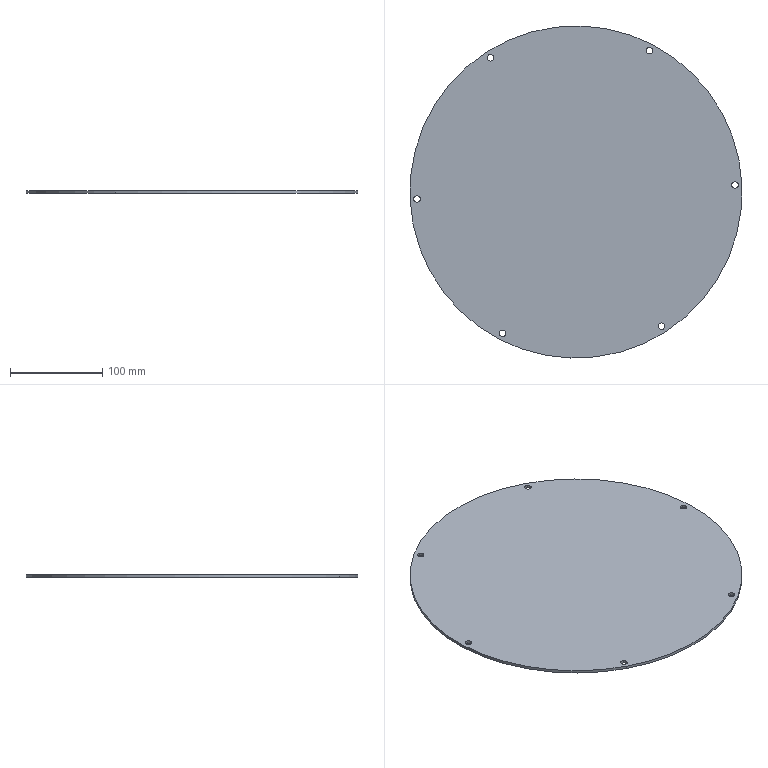Component | SolidWorks | YC1-250-02-21CrankshaftEndCover-1 | 1 solid | 16 faces | box 360 x 360 x 3 mm | volume 304670 mm3 | cylinder 14 | plane 2 | commonest cylinder face diameters 7 x12 360 x2 | material Plain Carbon Steel
STEP:
#1=COLOUR_RGB('',0.7922,0.8196,0.9333);
#2=FILL_AREA_STYLE_COLOUR('',#1);
#3=FILL_AREA_STYLE('',(#2));
#4=SURFACE_STYLE_FILL_AREA(#3);
#5=SURFACE_SIDE_STYLE('',(#4));
#6=SURFACE_STYLE_USAGE(.BOTH.,#5);
#7=PRESENTATION_STYLE_ASSIGNMENT((#6));
#8=CARTESIAN_POINT('',(-3.267,125.404,18.425));
#9=VERTEX_POINT('',#8);
#10=CARTESIAN_POINT('',(3.267,137.982,18.425));
#11=VERTEX_POINT('',#10);
#12=CARTESIAN_POINT('',(0.,131.693,18.425));
#13=DIRECTION('',(0.,0.,1.));
#14=DIRECTION('',(0.461,0.8874,0.));
#15=AXIS2_PLACEMENT_3D('',#12,#13,#14);
#16=CIRCLE('',#15,7.087);
#17=EDGE_CURVE('',#9,#11,#16,.T.);
#18=ORIENTED_EDGE('',*,*,#17,.F.);
#19=CARTESIAN_POINT('',(-3.267,125.404,18.307));
#20=VERTEX_POINT('',#19);
#21=CARTESIAN_POINT('',(-3.267,125.404,18.425));
#22=DIRECTION('',(0.,0.,-1.));
#23=VECTOR('',#22,39.37);
#24=LINE('',#21,#23);
#25=EDGE_CURVE('',#9,#20,#24,.T.);
#26=ORIENTED_EDGE('',*,*,#25,.T.);
#27=CARTESIAN_POINT('',(3.267,137.982,18.307));
#28=VERTEX_POINT('',#27);
#29=CARTESIAN_POINT('',(0.,131.693,18.307));
#30=DIRECTION('',(0.,0.,1.));
#31=DIRECTION('',(0.461,0.8874,0.));
#32=AXIS2_PLACEMENT_3D('',#29,#30,#31);
#33=CIRCLE('',#32,7.087);
#34=EDGE_CURVE('',#20,#28,#33,.T.);
#35=ORIENTED_EDGE('',*,*,#34,.T.);
#36=CARTESIAN_POINT('',(3.267,137.982,18.425));
#37=DIRECTION('',(0.,0.,-1.));
#38=VECTOR('',#37,39.37);
#39=LINE('',#36,#38);
#40=EDGE_CURVE('',#11,#28,#39,.T.);
#41=ORIENTED_EDGE('',*,*,#40,.F.);
#42=EDGE_LOOP('',(#18,#26,#35,#41));
#43=FACE_OUTER_BOUND('',#42,.T.);
#44=CARTESIAN_POINT('',(0.,131.693,18.425));
#45=DIRECTION('',(0.,0.,-1.));
#46=DIRECTION('',(0.461,0.8874,0.));
#47=AXIS2_PLACEMENT_3D('',#44,#45,#46);
#48=CYLINDRICAL_SURFACE('',#47,7.087);
#49=ADVANCED_FACE('',(#43),#48,.T.);
#50=CARTESIAN_POINT('',(-3.067,125.788,18.307));
#51=VERTEX_POINT('',#50);
#52=CARTESIAN_POINT('',(-3.194,125.544,18.307));
#53=VERTEX_POINT('',#52);
#54=CARTESIAN_POINT('',(-3.131,125.666,18.307));
#55=DIRECTION('',(0.,0.,1.));
#56=DIRECTION('',(-0.461,-0.8874,0.));
#57=AXIS2_PLACEMENT_3D('',#54,#55,#56);
#58=CIRCLE('',#57,0.1378);
#59=EDGE_CURVE('',#51,#53,#58,.T.);
#60=ORIENTED_EDGE('',*,*,#59,.F.);
#61=CARTESIAN_POINT('',(-3.067,125.788,18.425));
#62=VERTEX_POINT('',#61);
#63=CARTESIAN_POINT('',(-3.067,125.788,18.425));
#64=DIRECTION('',(0.,0.,1.));
#65=VECTOR('',#64,39.37);
#66=LINE('',#63,#65);
#67=EDGE_CURVE('',#51,#62,#66,.T.);
#68=ORIENTED_EDGE('',*,*,#67,.T.);
#69=CARTESIAN_POINT('',(-3.194,125.544,18.425));
#70=VERTEX_POINT('',#69);
#71=CARTESIAN_POINT('',(-3.131,125.666,18.425));
#72=DIRECTION('',(0.,0.,-1.));
#73=DIRECTION('',(-0.461,-0.8874,0.));
#74=AXIS2_PLACEMENT_3D('',#71,#72,#73);
#75=CIRCLE('',#74,0.1378);
#76=EDGE_CURVE('',#70,#62,#75,.T.);
#77=ORIENTED_EDGE('',*,*,#76,.F.);
#78=CARTESIAN_POINT('',(-3.194,125.544,18.425));
#79=DIRECTION('',(0.,0.,1.));
#80=VECTOR('',#79,39.37);
#81=LINE('',#78,#80);
#82=EDGE_CURVE('',#53,#70,#81,.T.);
#83=ORIENTED_EDGE('',*,*,#82,.F.);
#84=EDGE_LOOP('',(#60,#68,#77,#83));
#85=FACE_OUTER_BOUND('',#84,.T.);
#86=CARTESIAN_POINT('',(-3.131,125.666,18.425));
#87=DIRECTION('',(0.,0.,1.));
#88=DIRECTION('',(-0.461,-0.8874,0.));
#89=AXIS2_PLACEMENT_3D('',#86,#87,#88);
#90=CYLINDRICAL_SURFACE('',#89,0.1378);
#91=ADVANCED_FACE('',(#85),#90,.F.);
#92=CARTESIAN_POINT('',(-6.721,131.513,18.307));
#93=VERTEX_POINT('',#92);
#94=CARTESIAN_POINT('',(-6.848,131.268,18.307));
#95=VERTEX_POINT('',#94);
#96=CARTESIAN_POINT('',(-6.785,131.391,18.307));
#97=DIRECTION('',(0.,0.,1.));
#98=DIRECTION('',(-0.461,-0.8874,0.));
#99=AXIS2_PLACEMENT_3D('',#96,#97,#98);
#100=CIRCLE('',#99,0.1378);
#101=EDGE_CURVE('',#93,#95,#100,.T.);
#102=ORIENTED_EDGE('',*,*,#101,.F.);
#103=CARTESIAN_POINT('',(-6.721,131.513,18.425));
#104=VERTEX_POINT('',#103);
#105=CARTESIAN_POINT('',(-6.721,131.513,18.425));
#106=DIRECTION('',(0.,0.,1.));
#107=VECTOR('',#106,39.37);
#108=LINE('',#105,#107);
#109=EDGE_CURVE('',#93,#104,#108,.T.);
#110=ORIENTED_EDGE('',*,*,#109,.T.);
#111=CARTESIAN_POINT('',(-6.848,131.268,18.425));
#112=VERTEX_POINT('',#111);
#113=CARTESIAN_POINT('',(-6.785,131.391,18.425));
#114=DIRECTION('',(0.,0.,-1.));
#115=DIRECTION('',(-0.461,-0.8874,0.));
#116=AXIS2_PLACEMENT_3D('',#113,#114,#115);
#117=CIRCLE('',#116,0.1378);
#118=EDGE_CURVE('',#112,#104,#117,.T.);
#119=ORIENTED_EDGE('',*,*,#118,.F.);
#120=CARTESIAN_POINT('',(-6.848,131.268,18.425));
#121=DIRECTION('',(0.,0.,1.));
#122=VECTOR('',#121,39.37);
#123=LINE('',#120,#122);
#124=EDGE_CURVE('',#95,#112,#123,.T.);
#125=ORIENTED_EDGE('',*,*,#124,.F.);
#126=EDGE_LOOP('',(#102,#110,#119,#125));
#127=FACE_OUTER_BOUND('',#126,.T.);
#128=CARTESIAN_POINT('',(-6.785,131.391,18.425));
#129=DIRECTION('',(0.,0.,1.));
#130=DIRECTION('',(-0.461,-0.8874,0.));
#131=AXIS2_PLACEMENT_3D('',#128,#129,#130);
#132=CYLINDRICAL_SURFACE('',#131,0.1378);
#133=ADVANCED_FACE('',(#127),#132,.F.);
#134=CARTESIAN_POINT('',(-3.591,137.54,18.307));
#135=VERTEX_POINT('',#134);
#136=CARTESIAN_POINT('',(-3.718,137.295,18.307));
#137=VERTEX_POINT('',#136);
#138=CARTESIAN_POINT('',(-3.654,137.417,18.307));
#139=DIRECTION('',(0.,0.,1.));
#140=DIRECTION('',(-0.461,-0.8874,0.));
#141=AXIS2_PLACEMENT_3D('',#138,#139,#140);
#142=CIRCLE('',#141,0.1378);
#143=EDGE_CURVE('',#135,#137,#142,.T.);
#144=ORIENTED_EDGE('',*,*,#143,.F.);
#145=CARTESIAN_POINT('',(-3.591,137.54,18.425));
#146=VERTEX_POINT('',#145);
#147=CARTESIAN_POINT('',(-3.591,137.54,18.425));
#148=DIRECTION('',(0.,0.,1.));
#149=VECTOR('',#148,39.37);
#150=LINE('',#147,#149);
#151=EDGE_CURVE('',#135,#146,#150,.T.);
#152=ORIENTED_EDGE('',*,*,#151,.T.);
#153=CARTESIAN_POINT('',(-3.718,137.295,18.425));
#154=VERTEX_POINT('',#153);
#155=CARTESIAN_POINT('',(-3.654,137.417,18.425));
#156=DIRECTION('',(0.,0.,-1.));
#157=DIRECTION('',(-0.461,-0.8874,0.));
#158=AXIS2_PLACEMENT_3D('',#155,#156,#157);
#159=CIRCLE('',#158,0.1378);
#160=EDGE_CURVE('',#154,#146,#159,.T.);
#161=ORIENTED_EDGE('',*,*,#160,.F.);
#162=CARTESIAN_POINT('',(-3.718,137.295,18.425));
#163=DIRECTION('',(0.,0.,1.));
#164=VECTOR('',#163,39.37);
#165=LINE('',#162,#164);
#166=EDGE_CURVE('',#137,#154,#165,.T.);
#167=ORIENTED_EDGE('',*,*,#166,.F.);
#168=EDGE_LOOP('',(#144,#152,#161,#167));
#169=FACE_OUTER_BOUND('',#168,.T.);
#170=CARTESIAN_POINT('',(-3.654,137.417,18.425));
#171=DIRECTION('',(0.,0.,1.));
#172=DIRECTION('',(-0.461,-0.8874,0.));
#173=AXIS2_PLACEMENT_3D('',#170,#171,#172);
#174=CYLINDRICAL_SURFACE('',#173,0.1378);
#175=ADVANCED_FACE('',(#169),#174,.F.);
#176=CARTESIAN_POINT('',(3.194,137.842,18.307));
#177=VERTEX_POINT('',#176);
#178=CARTESIAN_POINT('',(3.067,137.597,18.307));
#179=VERTEX_POINT('',#178);
#180=CARTESIAN_POINT('',(3.131,137.72,18.307));
#181=DIRECTION('',(0.,0.,1.));
#182=DIRECTION('',(-0.461,-0.8874,0.));
#183=AXIS2_PLACEMENT_3D('',#180,#181,#182);
#184=CIRCLE('',#183,0.1378);
#185=EDGE_CURVE('',#177,#179,#184,.T.);
#186=ORIENTED_EDGE('',*,*,#185,.F.);
#187=CARTESIAN_POINT('',(3.194,137.842,18.425));
#188=VERTEX_POINT('',#187);
#189=CARTESIAN_POINT('',(3.194,137.842,18.425));
#190=DIRECTION('',(0.,0.,1.));
#191=VECTOR('',#190,39.37);
#192=LINE('',#189,#191);
#193=EDGE_CURVE('',#177,#188,#192,.T.);
#194=ORIENTED_EDGE('',*,*,#193,.T.);
#195=CARTESIAN_POINT('',(3.067,137.597,18.425));
#196=VERTEX_POINT('',#195);
#197=CARTESIAN_POINT('',(3.131,137.72,18.425));
#198=DIRECTION('',(0.,0.,-1.));
#199=DIRECTION('',(-0.461,-0.8874,0.));
#200=AXIS2_PLACEMENT_3D('',#197,#198,#199);
#201=CIRCLE('',#200,0.1378);
#202=EDGE_CURVE('',#196,#188,#201,.T.);
#203=ORIENTED_EDGE('',*,*,#202,.F.);
#204=CARTESIAN_POINT('',(3.067,137.597,18.425));
#205=DIRECTION('',(0.,0.,1.));
#206=VECTOR('',#205,39.37);
#207=LINE('',#204,#206);
#208=EDGE_CURVE('',#179,#196,#207,.T.);
#209=ORIENTED_EDGE('',*,*,#208,.F.);
#210=EDGE_LOOP('',(#186,#194,#203,#209));
#211=FACE_OUTER_BOUND('',#210,.T.);
#212=CARTESIAN_POINT('',(3.131,137.72,18.425));
#213=DIRECTION('',(0.,0.,1.));
#214=DIRECTION('',(-0.461,-0.8874,0.));
#215=AXIS2_PLACEMENT_3D('',#212,#213,#214);
#216=CYLINDRICAL_SURFACE('',#215,0.1378);
#217=ADVANCED_FACE('',(#211),#216,.F.);
#218=CARTESIAN_POINT('',(6.848,132.117,18.307));
#219=VERTEX_POINT('',#218);
#220=CARTESIAN_POINT('',(6.721,131.873,18.307));
#221=VERTEX_POINT('',#220);
#222=CARTESIAN_POINT('',(6.785,131.995,18.307));
#223=DIRECTION('',(0.,0.,1.));
#224=DIRECTION('',(-0.461,-0.8874,0.));
#225=AXIS2_PLACEMENT_3D('',#222,#223,#224);
#226=CIRCLE('',#225,0.1378);
#227=EDGE_CURVE('',#219,#221,#226,.T.);
#228=ORIENTED_EDGE('',*,*,#227,.F.);
#229=CARTESIAN_POINT('',(6.848,132.117,18.425));
#230=VERTEX_POINT('',#229);
#231=CARTESIAN_POINT('',(6.848,132.117,18.425));
#232=DIRECTION('',(0.,0.,1.));
#233=VECTOR('',#232,39.37);
#234=LINE('',#231,#233);
#235=EDGE_CURVE('',#219,#230,#234,.T.);
#236=ORIENTED_EDGE('',*,*,#235,.T.);
#237=CARTESIAN_POINT('',(6.721,131.873,18.425));
#238=VERTEX_POINT('',#237);
#239=CARTESIAN_POINT('',(6.785,131.995,18.425));
#240=DIRECTION('',(0.,0.,-1.));
#241=DIRECTION('',(-0.461,-0.8874,0.));
#242=AXIS2_PLACEMENT_3D('',#239,#240,#241);
#243=CIRCLE('',#242,0.1378);
#244=EDGE_CURVE('',#238,#230,#243,.T.);
#245=ORIENTED_EDGE('',*,*,#244,.F.);
#246=CARTESIAN_POINT('',(6.721,131.873,18.425));
#247=DIRECTION('',(0.,0.,1.));
#248=VECTOR('',#247,39.37);
#249=LINE('',#246,#248);
#250=EDGE_CURVE('',#221,#238,#249,.T.);
#251=ORIENTED_EDGE('',*,*,#250,.F.);
#252=EDGE_LOOP('',(#228,#236,#245,#251));
#253=FACE_OUTER_BOUND('',#252,.T.);
#254=CARTESIAN_POINT('',(6.785,131.995,18.425));
#255=DIRECTION('',(0.,0.,1.));
#256=DIRECTION('',(-0.461,-0.8874,0.));
#257=AXIS2_PLACEMENT_3D('',#254,#255,#256);
#258=CYLINDRICAL_SURFACE('',#257,0.1378);
#259=ADVANCED_FACE('',(#253),#258,.F.);
#260=CARTESIAN_POINT('',(3.718,126.091,18.307));
#261=VERTEX_POINT('',#260);
#262=CARTESIAN_POINT('',(3.591,125.846,18.307));
#263=VERTEX_POINT('',#262);
#264=CARTESIAN_POINT('',(3.654,125.968,18.307));
#265=DIRECTION('',(0.,0.,1.));
#266=DIRECTION('',(-0.461,-0.8874,0.));
#267=AXIS2_PLACEMENT_3D('',#264,#265,#266);
#268=CIRCLE('',#267,0.1378);
#269=EDGE_CURVE('',#261,#263,#268,.T.);
#270=ORIENTED_EDGE('',*,*,#269,.F.);
#271=CARTESIAN_POINT('',(3.718,126.091,18.425));
#272=VERTEX_POINT('',#271);
#273=CARTESIAN_POINT('',(3.718,126.091,18.425));
#274=DIRECTION('',(0.,0.,1.));
#275=VECTOR('',#274,39.37);
#276=LINE('',#273,#275);
#277=EDGE_CURVE('',#261,#272,#276,.T.);
#278=ORIENTED_EDGE('',*,*,#277,.T.);
#279=CARTESIAN_POINT('',(3.591,125.846,18.425));
#280=VERTEX_POINT('',#279);
#281=CARTESIAN_POINT('',(3.654,125.968,18.425));
#282=DIRECTION('',(0.,0.,-1.));
#283=DIRECTION('',(-0.461,-0.8874,0.));
#284=AXIS2_PLACEMENT_3D('',#281,#282,#283);
#285=CIRCLE('',#284,0.1378);
#286=EDGE_CURVE('',#280,#272,#285,.T.);
#287=ORIENTED_EDGE('',*,*,#286,.F.);
#288=CARTESIAN_POINT('',(3.591,125.846,18.425));
#289=DIRECTION('',(0.,0.,1.));
#290=VECTOR('',#289,39.37);
#291=LINE('',#288,#290);
#292=EDGE_CURVE('',#263,#280,#291,.T.);
#293=ORIENTED_EDGE('',*,*,#292,.F.);
#294=EDGE_LOOP('',(#270,#278,#287,#293));
#295=FACE_OUTER_BOUND('',#294,.T.);
#296=CARTESIAN_POINT('',(3.654,125.968,18.425));
#297=DIRECTION('',(0.,0.,1.));
#298=DIRECTION('',(-0.461,-0.8874,0.));
#299=AXIS2_PLACEMENT_3D('',#296,#297,#298);
#300=CYLINDRICAL_SURFACE('',#299,0.1378);
#301=ADVANCED_FACE('',(#295),#300,.F.);
#302=CARTESIAN_POINT('',(0.,131.693,18.425));
#303=DIRECTION('',(0.,0.,1.));
#304=DIRECTION('',(0.461,0.8874,0.));
#305=AXIS2_PLACEMENT_3D('',#302,#303,#304);
#306=CIRCLE('',#305,7.087);
#307=EDGE_CURVE('',#11,#9,#306,.T.);
#308=ORIENTED_EDGE('',*,*,#307,.T.);
#309=ORIENTED_EDGE('',*,*,#17,.T.);
#310=EDGE_LOOP('',(#308,#309));
#311=FACE_OUTER_BOUND('',#310,.T.);
#312=ORIENTED_EDGE('',*,*,#76,.T.);
#313=CARTESIAN_POINT('',(-3.131,125.666,18.425));
#314=DIRECTION('',(0.,0.,-1.));
#315=DIRECTION('',(-0.461,-0.8874,0.));
#316=AXIS2_PLACEMENT_3D('',#313,#314,#315);
#317=CIRCLE('',#316,0.1378);
#318=EDGE_CURVE('',#62,#70,#317,.T.);
#319=ORIENTED_EDGE('',*,*,#318,.T.);
#320=EDGE_LOOP('',(#312,#319));
#321=FACE_BOUND('',#320,.T.);
#322=ORIENTED_EDGE('',*,*,#118,.T.);
#323=CARTESIAN_POINT('',(-6.785,131.391,18.425));
#324=DIRECTION('',(0.,0.,-1.));
#325=DIRECTION('',(-0.461,-0.8874,0.));
#326=AXIS2_PLACEMENT_3D('',#323,#324,#325);
#327=CIRCLE('',#326,0.1378);
#328=EDGE_CURVE('',#104,#112,#327,.T.);
#329=ORIENTED_EDGE('',*,*,#328,.T.);
#330=EDGE_LOOP('',(#322,#329));
#331=FACE_BOUND('',#330,.T.);
#332=ORIENTED_EDGE('',*,*,#160,.T.);
#333=CARTESIAN_POINT('',(-3.654,137.417,18.425));
#334=DIRECTION('',(0.,0.,-1.));
#335=DIRECTION('',(-0.461,-0.8874,0.));
#336=AXIS2_PLACEMENT_3D('',#333,#334,#335);
#337=CIRCLE('',#336,0.1378);
#338=EDGE_CURVE('',#146,#154,#337,.T.);
#339=ORIENTED_EDGE('',*,*,#338,.T.);
#340=EDGE_LOOP('',(#332,#339));
#341=FACE_BOUND('',#340,.T.);
#342=ORIENTED_EDGE('',*,*,#202,.T.);
#343=CARTESIAN_POINT('',(3.131,137.72,18.425));
#344=DIRECTION('',(0.,0.,-1.));
#345=DIRECTION('',(-0.461,-0.8874,0.));
#346=AXIS2_PLACEMENT_3D('',#343,#344,#345);
#347=CIRCLE('',#346,0.1378);
#348=EDGE_CURVE('',#188,#196,#347,.T.);
#349=ORIENTED_EDGE('',*,*,#348,.T.);
#350=EDGE_LOOP('',(#342,#349));
#351=FACE_BOUND('',#350,.T.);
#352=ORIENTED_EDGE('',*,*,#244,.T.);
#353=CARTESIAN_POINT('',(6.785,131.995,18.425));
#354=DIRECTION('',(0.,0.,-1.));
#355=DIRECTION('',(-0.461,-0.8874,0.));
#356=AXIS2_PLACEMENT_3D('',#353,#354,#355);
#357=CIRCLE('',#356,0.1378);
#358=EDGE_CURVE('',#230,#238,#357,.T.);
#359=ORIENTED_EDGE('',*,*,#358,.T.);
#360=EDGE_LOOP('',(#352,#359));
#361=FACE_BOUND('',#360,.T.);
#362=ORIENTED_EDGE('',*,*,#286,.T.);
#363=CARTESIAN_POINT('',(3.654,125.968,18.425));
#364=DIRECTION('',(0.,0.,-1.));
#365=DIRECTION('',(-0.461,-0.8874,0.));
#366=AXIS2_PLACEMENT_3D('',#363,#364,#365);
#367=CIRCLE('',#366,0.1378);
#368=EDGE_CURVE('',#272,#280,#367,.T.);
#369=ORIENTED_EDGE('',*,*,#368,.T.);
#370=EDGE_LOOP('',(#362,#369));
#371=FACE_BOUND('',#370,.T.);
#372=CARTESIAN_POINT('',(0.,131.693,18.425));
#373=DIRECTION('',(0.,0.,1.));
#374=DIRECTION('',(-0.461,-0.8874,0.));
#375=AXIS2_PLACEMENT_3D('',#372,#373,#374);
#376=PLANE('',#375);
#377=ADVANCED_FACE('',(#311,#321,#331,#341,#351,#361,#371),#376,.T.);
#378=ORIENTED_EDGE('',*,*,#25,.F.);
#379=ORIENTED_EDGE('',*,*,#307,.F.);
#380=ORIENTED_EDGE('',*,*,#40,.T.);
#381=CARTESIAN_POINT('',(0.,131.693,18.307));
#382=DIRECTION('',(0.,0.,1.));
#383=DIRECTION('',(0.461,0.8874,0.));
#384=AXIS2_PLACEMENT_3D('',#381,#382,#383);
#385=CIRCLE('',#384,7.087);
#386=EDGE_CURVE('',#28,#20,#385,.T.);
#387=ORIENTED_EDGE('',*,*,#386,.T.);
#388=EDGE_LOOP('',(#378,#379,#380,#387));
#389=FACE_OUTER_BOUND('',#388,.T.);
#390=CARTESIAN_POINT('',(0.,131.693,18.425));
#391=DIRECTION('',(0.,0.,-1.));
#392=DIRECTION('',(0.461,0.8874,0.));
#393=AXIS2_PLACEMENT_3D('',#390,#391,#392);
#394=CYLINDRICAL_SURFACE('',#393,7.087);
#395=ADVANCED_FACE('',(#389),#394,.T.);
#396=ORIENTED_EDGE('',*,*,#67,.F.);
#397=CARTESIAN_POINT('',(-3.131,125.666,18.307));
#398=DIRECTION('',(0.,0.,1.));
#399=DIRECTION('',(-0.461,-0.8874,0.));
#400=AXIS2_PLACEMENT_3D('',#397,#398,#399);
#401=CIRCLE('',#400,0.1378);
#402=EDGE_CURVE('',#53,#51,#401,.T.);
#403=ORIENTED_EDGE('',*,*,#402,.F.);
#404=ORIENTED_EDGE('',*,*,#82,.T.);
#405=ORIENTED_EDGE('',*,*,#318,.F.);
#406=EDGE_LOOP('',(#396,#403,#404,#405));
#407=FACE_OUTER_BOUND('',#406,.T.);
#408=CARTESIAN_POINT('',(-3.131,125.666,18.425));
#409=DIRECTION('',(0.,0.,1.));
#410=DIRECTION('',(-0.461,-0.8874,0.));
#411=AXIS2_PLACEMENT_3D('',#408,#409,#410);
#412=CYLINDRICAL_SURFACE('',#411,0.1378);
#413=ADVANCED_FACE('',(#407),#412,.F.);
#414=ORIENTED_EDGE('',*,*,#109,.F.);
#415=CARTESIAN_POINT('',(-6.785,131.391,18.307));
#416=DIRECTION('',(0.,0.,1.));
#417=DIRECTION('',(-0.461,-0.8874,0.));
#418=AXIS2_PLACEMENT_3D('',#415,#416,#417);
#419=CIRCLE('',#418,0.1378);
#420=EDGE_CURVE('',#95,#93,#419,.T.);
#421=ORIENTED_EDGE('',*,*,#420,.F.);
#422=ORIENTED_EDGE('',*,*,#124,.T.);
#423=ORIENTED_EDGE('',*,*,#328,.F.);
#424=EDGE_LOOP('',(#414,#421,#422,#423));
#425=FACE_OUTER_BOUND('',#424,.T.);
#426=CARTESIAN_POINT('',(-6.785,131.391,18.425));
#427=DIRECTION('',(0.,0.,1.));
#428=DIRECTION('',(-0.461,-0.8874,0.));
#429=AXIS2_PLACEMENT_3D('',#426,#427,#428);
#430=CYLINDRICAL_SURFACE('',#429,0.1378);
#431=ADVANCED_FACE('',(#425),#430,.F.);
#432=ORIENTED_EDGE('',*,*,#151,.F.);
#433=CARTESIAN_POINT('',(-3.654,137.417,18.307));
#434=DIRECTION('',(0.,0.,1.));
#435=DIRECTION('',(-0.461,-0.8874,0.));
#436=AXIS2_PLACEMENT_3D('',#433,#434,#435);
#437=CIRCLE('',#436,0.1378);
#438=EDGE_CURVE('',#137,#135,#437,.T.);
#439=ORIENTED_EDGE('',*,*,#438,.F.);
#440=ORIENTED_EDGE('',*,*,#166,.T.);
#441=ORIENTED_EDGE('',*,*,#338,.F.);
#442=EDGE_LOOP('',(#432,#439,#440,#441));
#443=FACE_OUTER_BOUND('',#442,.T.);
#444=CARTESIAN_POINT('',(-3.654,137.417,18.425));
#445=DIRECTION('',(0.,0.,1.));
#446=DIRECTION('',(-0.461,-0.8874,0.));
#447=AXIS2_PLACEMENT_3D('',#444,#445,#446);
#448=CYLINDRICAL_SURFACE('',#447,0.1378);
#449=ADVANCED_FACE('',(#443),#448,.F.);
#450=ORIENTED_EDGE('',*,*,#193,.F.);
#451=CARTESIAN_POINT('',(3.131,137.72,18.307));
#452=DIRECTION('',(0.,0.,1.));
#453=DIRECTION('',(-0.461,-0.8874,0.));
#454=AXIS2_PLACEMENT_3D('',#451,#452,#453);
#455=CIRCLE('',#454,0.1378);
#456=EDGE_CURVE('',#179,#177,#455,.T.);
#457=ORIENTED_EDGE('',*,*,#456,.F.);
#458=ORIENTED_EDGE('',*,*,#208,.T.);
#459=ORIENTED_EDGE('',*,*,#348,.F.);
#460=EDGE_LOOP('',(#450,#457,#458,#459));
#461=FACE_OUTER_BOUND('',#460,.T.);
#462=CARTESIAN_POINT('',(3.131,137.72,18.425));
#463=DIRECTION('',(0.,0.,1.));
#464=DIRECTION('',(-0.461,-0.8874,0.));
#465=AXIS2_PLACEMENT_3D('',#462,#463,#464);
#466=CYLINDRICAL_SURFACE('',#465,0.1378);
#467=ADVANCED_FACE('',(#461),#466,.F.);
#468=ORIENTED_EDGE('',*,*,#235,.F.);
#469=CARTESIAN_POINT('',(6.785,131.995,18.307));
#470=DIRECTION('',(0.,0.,1.));
#471=DIRECTION('',(-0.461,-0.8874,0.));
#472=AXIS2_PLACEMENT_3D('',#469,#470,#471);
#473=CIRCLE('',#472,0.1378);
#474=EDGE_CURVE('',#221,#219,#473,.T.);
#475=ORIENTED_EDGE('',*,*,#474,.F.);
#476=ORIENTED_EDGE('',*,*,#250,.T.);
#477=ORIENTED_EDGE('',*,*,#358,.F.);
#478=EDGE_LOOP('',(#468,#475,#476,#477));
#479=FACE_OUTER_BOUND('',#478,.T.);
#480=CARTESIAN_POINT('',(6.785,131.995,18.425));
#481=DIRECTION('',(0.,0.,1.));
#482=DIRECTION('',(-0.461,-0.8874,0.));
#483=AXIS2_PLACEMENT_3D('',#480,#481,#482);
#484=CYLINDRICAL_SURFACE('',#483,0.1378);
#485=ADVANCED_FACE('',(#479),#484,.F.);
#486=ORIENTED_EDGE('',*,*,#277,.F.);
#487=CARTESIAN_POINT('',(3.654,125.968,18.307));
#488=DIRECTION('',(0.,0.,1.));
#489=DIRECTION('',(-0.461,-0.8874,0.));
#490=AXIS2_PLACEMENT_3D('',#487,#488,#489);
#491=CIRCLE('',#490,0.1378);
#492=EDGE_CURVE('',#263,#261,#491,.T.);
#493=ORIENTED_EDGE('',*,*,#492,.F.);
#494=ORIENTED_EDGE('',*,*,#292,.T.);
#495=ORIENTED_EDGE('',*,*,#368,.F.);
#496=EDGE_LOOP('',(#486,#493,#494,#495));
#497=FACE_OUTER_BOUND('',#496,.T.);
#498=CARTESIAN_POINT('',(3.654,125.968,18.425));
#499=DIRECTION('',(0.,0.,1.));
#500=DIRECTION('',(-0.461,-0.8874,0.));
#501=AXIS2_PLACEMENT_3D('',#498,#499,#500);
#502=CYLINDRICAL_SURFACE('',#501,0.1378);
#503=ADVANCED_FACE('',(#497),#502,.F.);
#504=ORIENTED_EDGE('',*,*,#386,.F.);
#505=ORIENTED_EDGE('',*,*,#34,.F.);
#506=EDGE_LOOP('',(#504,#505));
#507=FACE_OUTER_BOUND('',#506,.T.);
#508=ORIENTED_EDGE('',*,*,#402,.T.);
#509=ORIENTED_EDGE('',*,*,#59,.T.);
#510=EDGE_LOOP('',(#508,#509));
#511=FACE_BOUND('',#510,.T.);
#512=ORIENTED_EDGE('',*,*,#420,.T.);
#513=ORIENTED_EDGE('',*,*,#101,.T.);
#514=EDGE_LOOP('',(#512,#513));
#515=FACE_BOUND('',#514,.T.);
#516=ORIENTED_EDGE('',*,*,#438,.T.);
#517=ORIENTED_EDGE('',*,*,#143,.T.);
#518=EDGE_LOOP('',(#516,#517));
#519=FACE_BOUND('',#518,.T.);
#520=ORIENTED_EDGE('',*,*,#456,.T.);
#521=ORIENTED_EDGE('',*,*,#185,.T.);
#522=EDGE_LOOP('',(#520,#521));
#523=FACE_BOUND('',#522,.T.);
#524=ORIENTED_EDGE('',*,*,#474,.T.);
#525=ORIENTED_EDGE('',*,*,#227,.T.);
#526=EDGE_LOOP('',(#524,#525));
#527=FACE_BOUND('',#526,.T.);
#528=ORIENTED_EDGE('',*,*,#492,.T.);
#529=ORIENTED_EDGE('',*,*,#269,.T.);
#530=EDGE_LOOP('',(#528,#529));
#531=FACE_BOUND('',#530,.T.);
#532=CARTESIAN_POINT('',(0.,131.693,18.307));
#533=DIRECTION('',(0.,0.,1.));
#534=DIRECTION('',(-0.461,-0.8874,0.));
#535=AXIS2_PLACEMENT_3D('',#532,#533,#534);
#536=PLANE('',#535);
#537=ADVANCED_FACE('',(#507,#511,#515,#519,#523,#527,#531),#536,.F.);
#538=CLOSED_SHELL('',(#49,#91,#133,#175,#217,#259,#301,#377,#395,#413,#431,#449,#467,#485,#503,#537));
#539=MANIFOLD_SOLID_BREP('',#538);
#540=STYLED_ITEM('',(#7),#539);
#541=PRESENTATION_LAYER_ASSIGNMENT('','',(#540));
#542=(LENGTH_UNIT()NAMED_UNIT(*)SI_UNIT($,.METRE.));
#543=LENGTH_MEASURE_WITH_UNIT(LENGTH_MEASURE(0.0254),#542);
#544=DIMENSIONAL_EXPONENTS(1.,0.,0.,0.,0.,0.,0.);
#545=(CONVERSION_BASED_UNIT('',#543)LENGTH_UNIT()NAMED_UNIT(#544));
#546=UNCERTAINTY_MEASURE_WITH_UNIT(LENGTH_MEASURE(0.00001),#545,'','');
#547=(NAMED_UNIT(*)PLANE_ANGLE_UNIT()SI_UNIT($,.RADIAN.));
#548=(NAMED_UNIT(*)SI_UNIT($,.STERADIAN.)SOLID_ANGLE_UNIT());
#549=(GEOMETRIC_REPRESENTATION_CONTEXT(3)GLOBAL_UNCERTAINTY_ASSIGNED_CONTEXT((#546))GLOBAL_UNIT_ASSIGNED_CONTEXT((#545,#547,#548))REPRESENTATION_CONTEXT('',''));
#550=MECHANICAL_DESIGN_GEOMETRIC_PRESENTATION_REPRESENTATION('',(#540),#549);
#551=CARTESIAN_POINT('',(0.,0.,0.));
#552=DIRECTION('',(0.,0.,1.));
#553=DIRECTION('',(1.,0.,0.));
#554=AXIS2_PLACEMENT_3D('',#551,#552,#553);
#555=(LENGTH_UNIT()NAMED_UNIT(*)SI_UNIT($,.METRE.));
#556=LENGTH_MEASURE_WITH_UNIT(LENGTH_MEASURE(0.0254),#555);
#557=DIMENSIONAL_EXPONENTS(1.,0.,0.,0.,0.,0.,0.);
#558=(CONVERSION_BASED_UNIT('',#556)LENGTH_UNIT()NAMED_UNIT(#557));
#559=UNCERTAINTY_MEASURE_WITH_UNIT(LENGTH_MEASURE(0.00001),#558,'','');
#560=(NAMED_UNIT(*)PLANE_ANGLE_UNIT()SI_UNIT($,.RADIAN.));
#561=(NAMED_UNIT(*)SI_UNIT($,.STERADIAN.)SOLID_ANGLE_UNIT());
#562=(GEOMETRIC_REPRESENTATION_CONTEXT(3)GLOBAL_UNCERTAINTY_ASSIGNED_CONTEXT((#559))GLOBAL_UNIT_ASSIGNED_CONTEXT((#558,#560,#561))REPRESENTATION_CONTEXT('',''));
#563=ADVANCED_BREP_SHAPE_REPRESENTATION('',(#539,#554),#562);